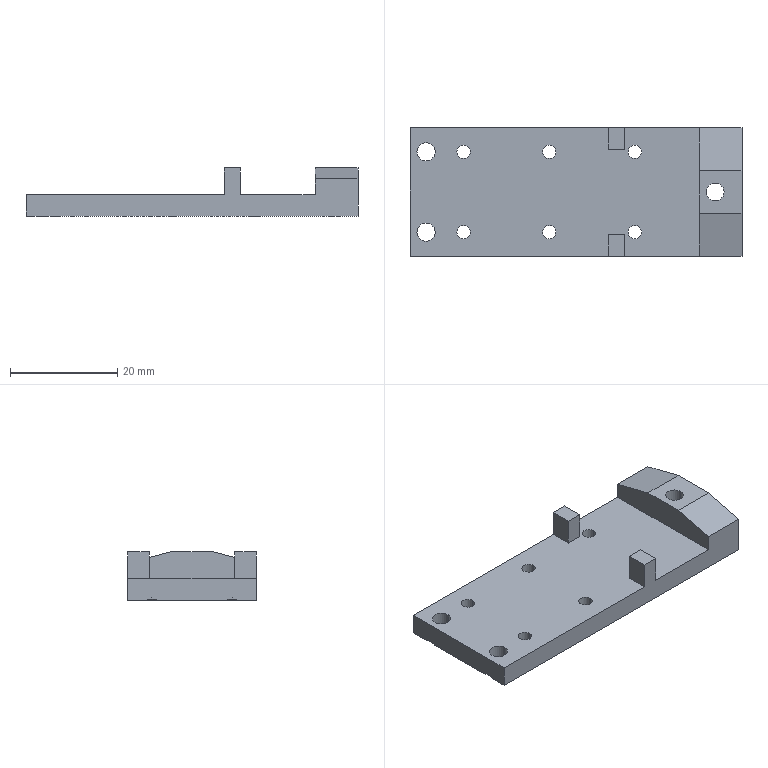Component | SolidWorks | JR-PL-JD-03BasePlate-1 | 1 solid | 52 faces | box 62 x 24 x 9 mm | volume 6602 mm3 | cylinder 18 | plane 18 | cone 16 | commonest cylinder face diameters 2.5 x12 3.4 x4 3.3 x2
build123d program:
from build123d import *

# Parameters (mm, degrees)
SKETCH1_W                                            = 62
SKETCH1_H                                            = 24
BOSS_EXTRUDE1_DEPTH                                  = 4
SKETCH4_W                                            = 8
SKETCH4_H                                            = 24
BOSS_EXTRUDE2_DEPTH                                  = 5
M4_TAPPED_HOLE1_D                                    = 3.3
CUT_EXTRUDE1_DEPTH                                   = 68.089
SKETCH6_W                                            = 3
SKETCH6_H                                            = 4
BOSS_EXTRUDE3_DEPTH                                  = 5
HOLE_SIZE_SLOTTED_RAISED_COUNTERSUNK_SCR_D           = 3.4
HOLE_SIZE_SLOTTED_RAISED_COUNTERSUNK_SCR_DEPTH       = 8.5
HOLE_SIZE_SLOTTED_RAISED_COUNTERSUNK_SCR_CSINK_D     = 6.4
HOLE_SIZE_SLOTTED_RAISED_COUNTERSUNK_SCR_CSINK_ANGLE = 90
HOLE_SIZE_SLOTTED_RAISED_COUNTERSUNK_SCR_TIP         = 1.021
M3_TAPPED_HOLE1_D                                    = 2.5
M3_TAPPED_HOLE1_CSINK_D                              = 3.05
M3_TAPPED_HOLE1_CSINK_ANGLE                          = 90


with BuildPart() as part:
    # Sketch1 → Boss-Extrude1 (new body)
    with BuildSketch(Plane.XY):
        with Locations((31, 12)):
            Rectangle(SKETCH1_W, SKETCH1_H)
    extrude(amount=BOSS_EXTRUDE1_DEPTH)

    # Sketch4 → Boss-Extrude2 (add)
    with BuildSketch(Plane.XY.offset(4)):
        with Locations((58, 12)):
            Rectangle(SKETCH4_W, SKETCH4_H)
    extrude(amount=BOSS_EXTRUDE2_DEPTH)

    # M4 Tapped Hole1 (through all)
    with Locations(Plane(origin=(0, 0, 0), x_dir=(1, 0, 0), z_dir=(0, 0, -1))):
        with Locations((57, -12)):
            Hole(M4_TAPPED_HOLE1_D / 2)

    # Sketch5 → Cut-Extrude1 (cut, through all)
    with BuildSketch(Plane(origin=(62, 0, 0), x_dir=(0, 0, -1), z_dir=(1, 0, 0))):
        Polygon((-9, 8), (-6.974, 0), (-9, 0), align=None)
        Polygon((-9, 24), (-9, 16), (-6.974, 24), align=None)
    extrude(amount=-CUT_EXTRUDE1_DEPTH, mode=Mode.SUBTRACT)

    # Sketch6 → Boss-Extrude3 (add)
    with BuildSketch(Plane.XY.offset(4)):
        with Locations((38.5, 22)):
            Rectangle(SKETCH6_W, SKETCH6_H)
        with Locations((38.5, 2)):
            Rectangle(SKETCH6_W, SKETCH6_H)
    extrude(amount=BOSS_EXTRUDE3_DEPTH)

    # Hole Size Slotted Raised Countersunk Scr
    with Locations(Plane(origin=(0, 0, 0), x_dir=(-1, 0, 0), z_dir=(0, 0, -1))):
        with Locations((-3, 4.5), (-3, 19.5)):
            CounterSinkHole(HOLE_SIZE_SLOTTED_RAISED_COUNTERSUNK_SCR_D / 2, HOLE_SIZE_SLOTTED_RAISED_COUNTERSUNK_SCR_CSINK_D / 2, depth=HOLE_SIZE_SLOTTED_RAISED_COUNTERSUNK_SCR_DEPTH, counter_sink_angle=HOLE_SIZE_SLOTTED_RAISED_COUNTERSUNK_SCR_CSINK_ANGLE)
            with Locations((0, 0, -(HOLE_SIZE_SLOTTED_RAISED_COUNTERSUNK_SCR_DEPTH + HOLE_SIZE_SLOTTED_RAISED_COUNTERSUNK_SCR_TIP / 2))):  # 118° drill point
                Cone(0, HOLE_SIZE_SLOTTED_RAISED_COUNTERSUNK_SCR_D / 2, HOLE_SIZE_SLOTTED_RAISED_COUNTERSUNK_SCR_TIP, mode=Mode.SUBTRACT)

    # M3 Tapped Hole1 (through all)
    with Locations(Plane(origin=(0, 0, 0), x_dir=(-1, 0, 0), z_dir=(0, 0, -1))):
        with Locations((-42, 19.5), (-42, 4.5), (-26, 19.5), (-26, 4.5), (-10, 19.5), (-10, 4.5)):
            CounterSinkHole(M3_TAPPED_HOLE1_D / 2, M3_TAPPED_HOLE1_CSINK_D / 2, counter_sink_angle=M3_TAPPED_HOLE1_CSINK_ANGLE)


solid = part.part

# Placed as in the assembly
solid = solid.moved(Location((-19.325, 18.452, 58.77), (0, 0, 0)))